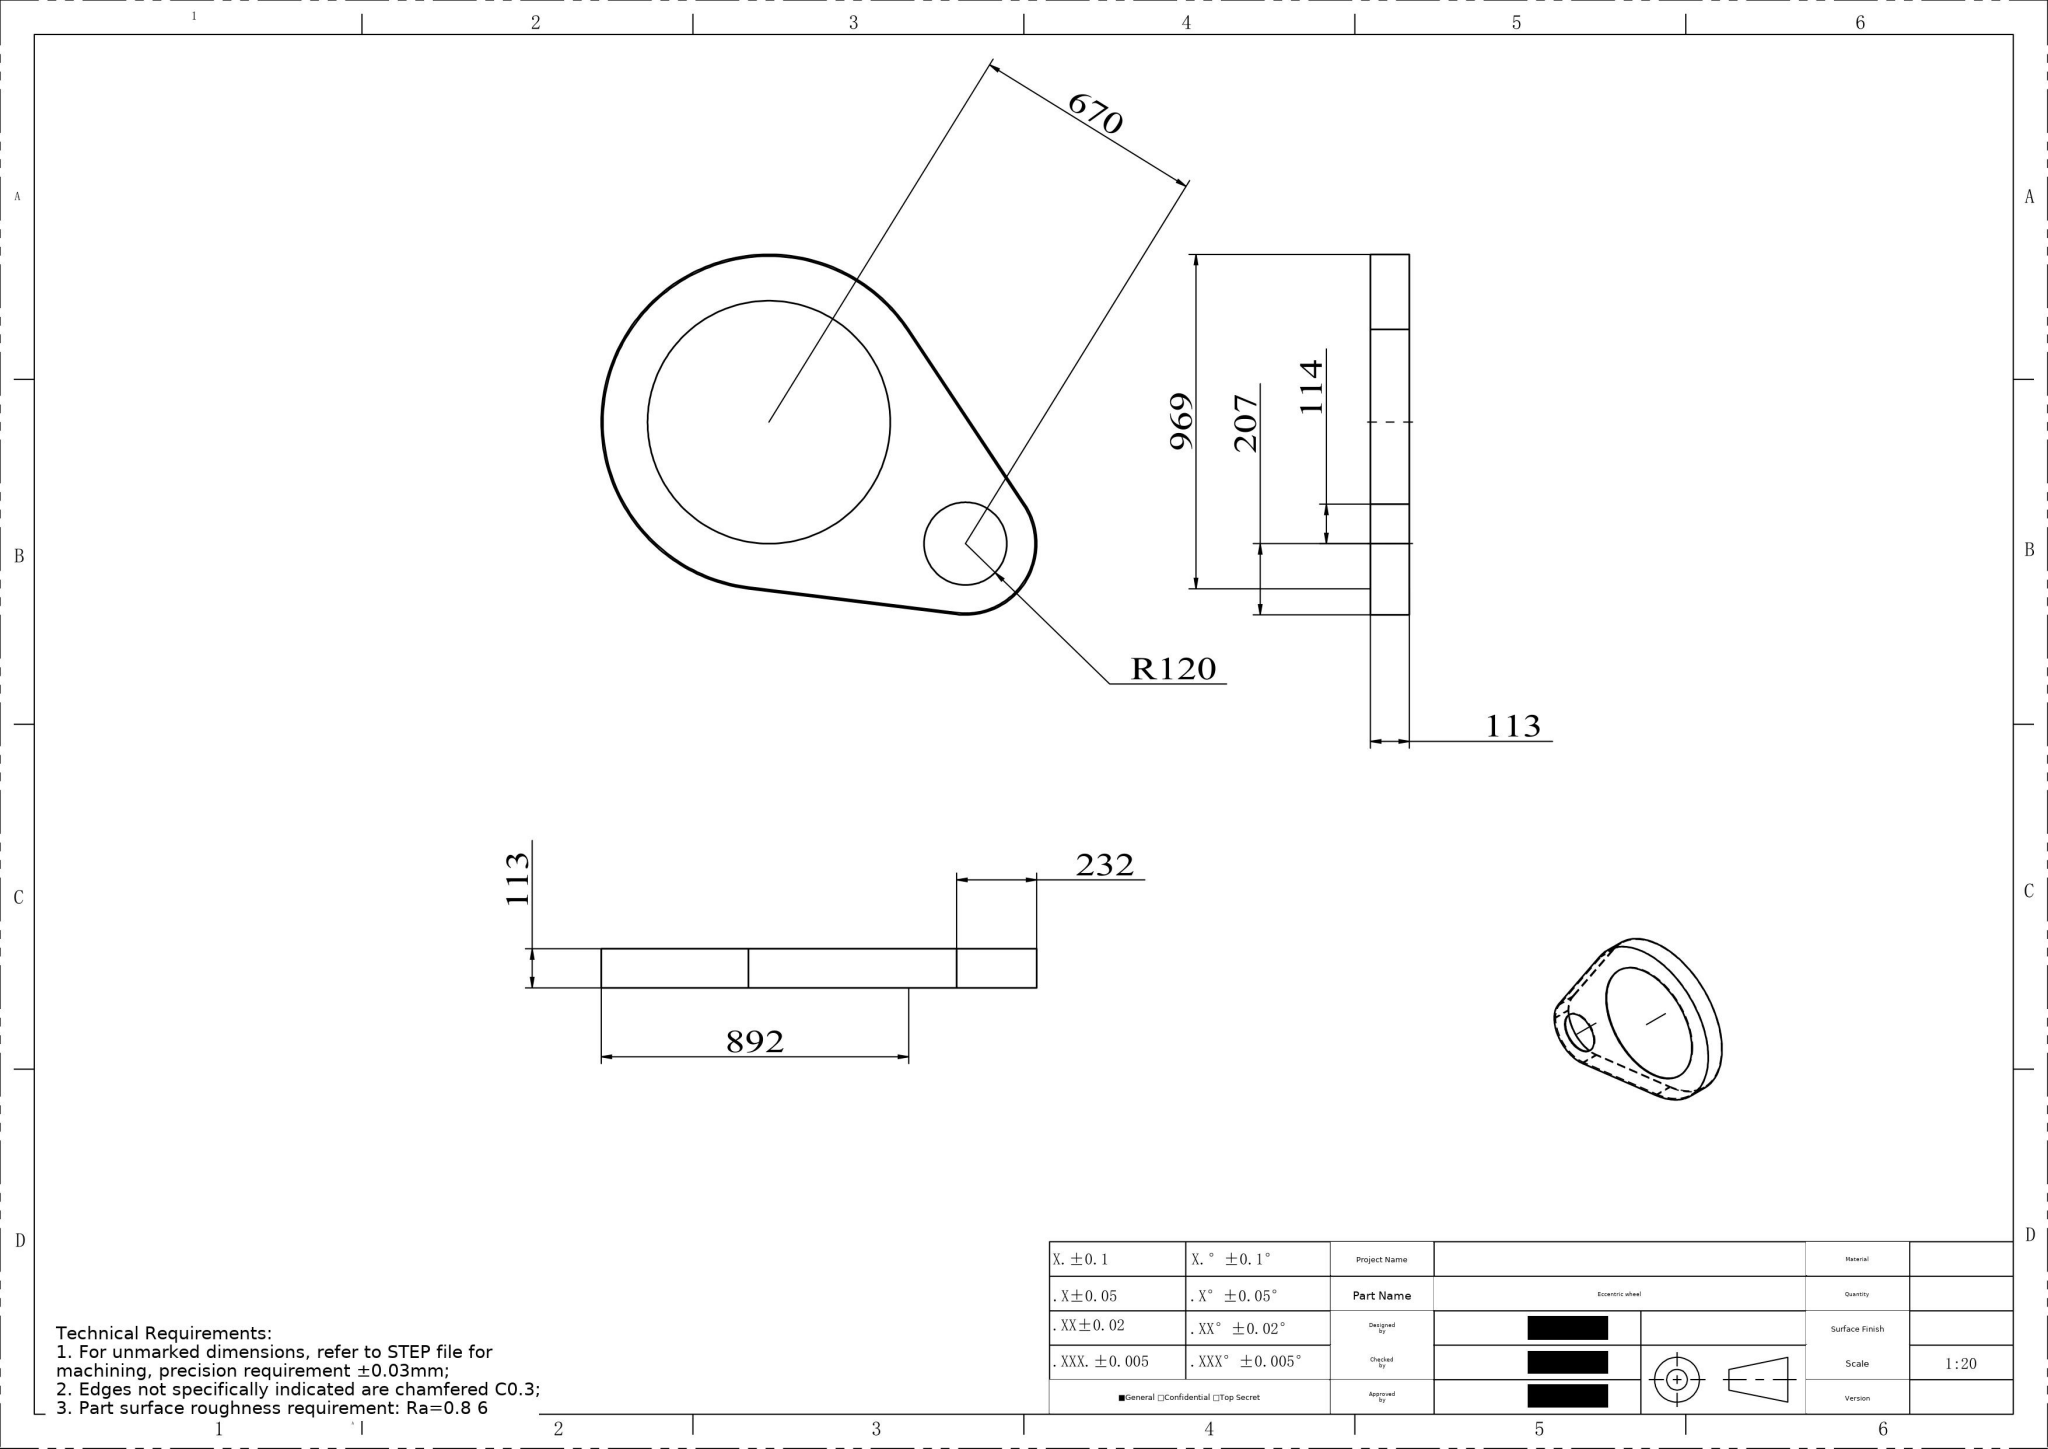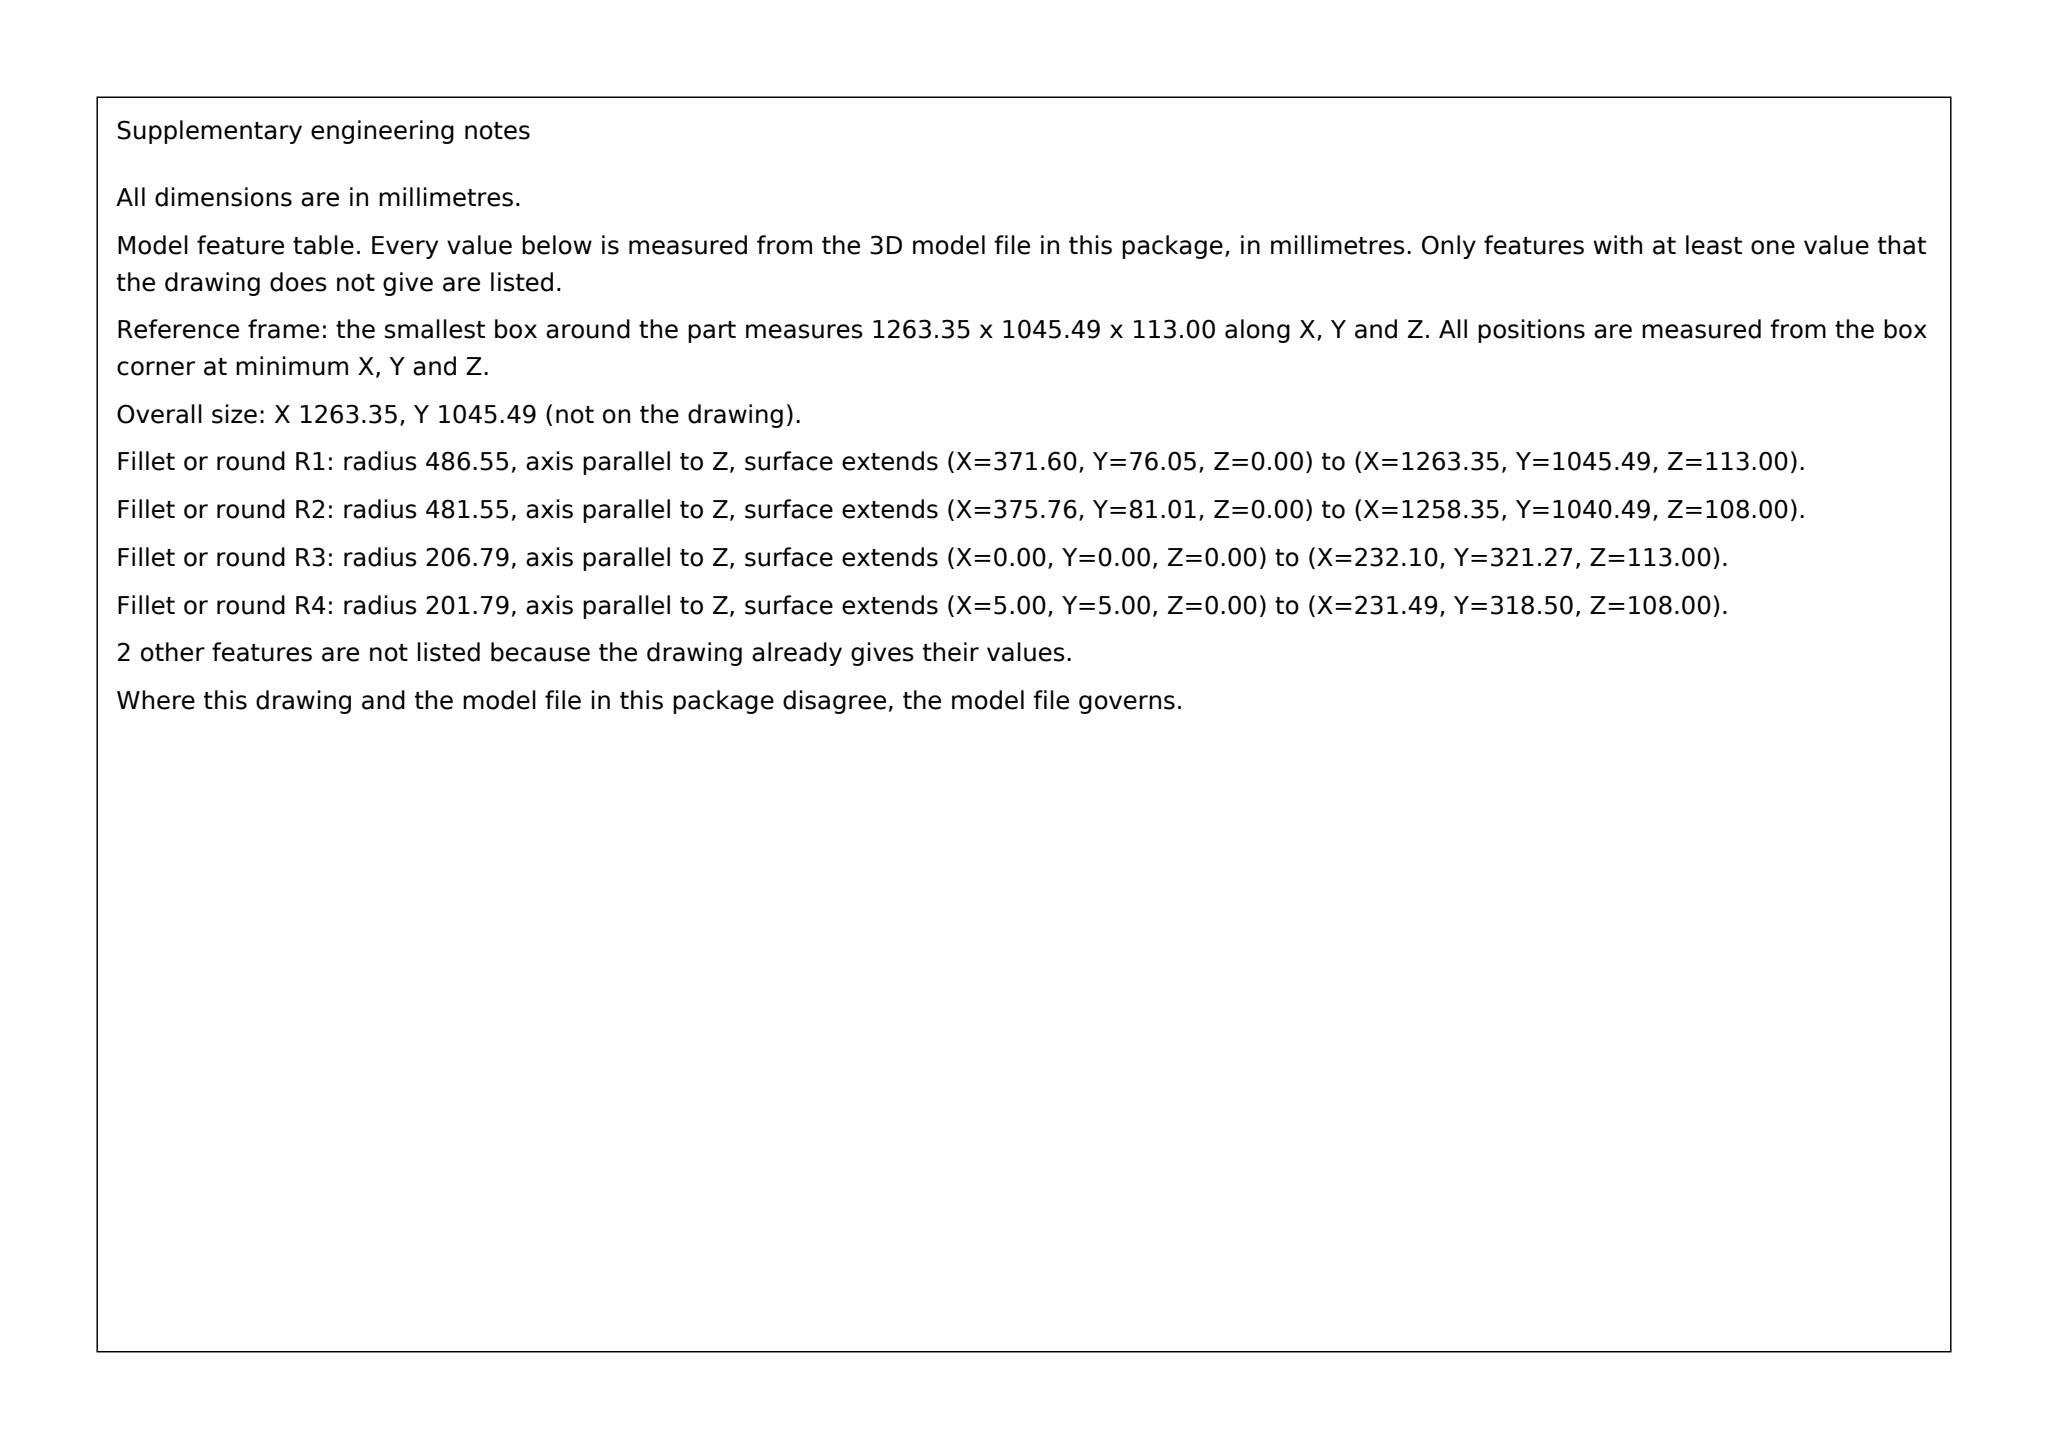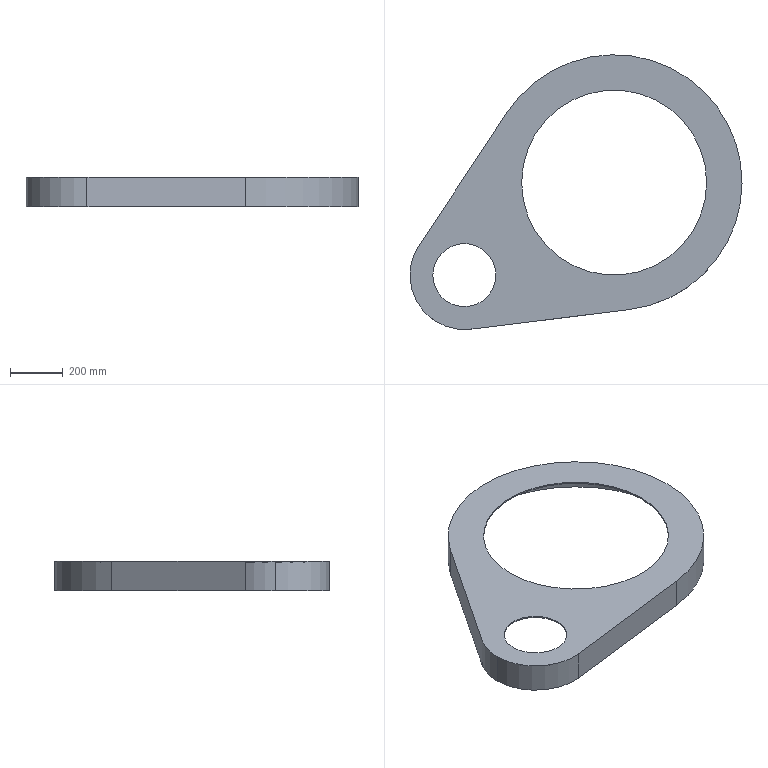Part | SolidWorks | mm | 1 solid | 17 faces | box 1263.35 x 1045.49 x 113 mm | volume 4506392 mm3 | cylinder 10 | plane 7 | commonest cylinder face diameters 240 x2 704 x2 403.589 x2 413.589 x2 963.102 x1 973.102 x1
STEP:
#1=CARTESIAN_POINT('',(-641.923,501.103,891.033));
#2=VERTEX_POINT('',#1);
#3=CARTESIAN_POINT('',(-641.923,501.103,886.033));
#4=VERTEX_POINT('',#3);
#5=CARTESIAN_POINT('',(-641.923,501.103,886.033));
#6=DIRECTION('',(0.,0.,-1.));
#7=VECTOR('',#6,1000.);
#8=LINE('',#5,#7);
#9=EDGE_CURVE('',#2,#4,#8,.T.);
#10=ORIENTED_EDGE('',*,*,#9,.F.);
#11=CARTESIAN_POINT('',(-881.923,501.103,891.033));
#12=VERTEX_POINT('',#11);
#13=CARTESIAN_POINT('',(-761.923,501.103,891.033));
#14=DIRECTION('',(0.,0.,-1.));
#15=DIRECTION('',(-1.,0.,0.));
#16=AXIS2_PLACEMENT_3D('',#13,#14,#15);
#17=CIRCLE('',#16,120.);
#18=EDGE_CURVE('',#12,#2,#17,.T.);
#19=ORIENTED_EDGE('',*,*,#18,.F.);
#20=CARTESIAN_POINT('',(-881.923,501.103,886.033));
#21=VERTEX_POINT('',#20);
#22=CARTESIAN_POINT('',(-881.923,501.103,886.033));
#23=DIRECTION('',(0.,0.,-1.));
#24=VECTOR('',#23,1000.);
#25=LINE('',#22,#24);
#26=EDGE_CURVE('',#12,#21,#25,.T.);
#27=ORIENTED_EDGE('',*,*,#26,.T.);
#28=CARTESIAN_POINT('',(-761.923,501.103,886.033));
#29=DIRECTION('',(0.,0.,-1.));
#30=DIRECTION('',(-1.,0.,0.));
#31=AXIS2_PLACEMENT_3D('',#28,#29,#30);
#32=CIRCLE('',#31,120.);
#33=EDGE_CURVE('',#21,#4,#32,.T.);
#34=ORIENTED_EDGE('',*,*,#33,.T.);
#35=EDGE_LOOP('',(#10,#19,#27,#34));
#36=FACE_OUTER_BOUND('',#35,.T.);
#37=CARTESIAN_POINT('',(-761.923,501.103,886.033));
#38=DIRECTION('',(0.,0.,-1.));
#39=DIRECTION('',(-1.,0.,0.));
#40=AXIS2_PLACEMENT_3D('',#37,#38,#39);
#41=CYLINDRICAL_SURFACE('',#40,120.);
#42=ADVANCED_FACE('',(#36),#41,.F.);
#43=CARTESIAN_POINT('',(160.077,853.249,891.033));
#44=VERTEX_POINT('',#43);
#45=CARTESIAN_POINT('',(160.077,853.249,886.033));
#46=VERTEX_POINT('',#45);
#47=CARTESIAN_POINT('',(160.077,853.249,886.033));
#48=DIRECTION('',(0.,0.,-1.));
#49=VECTOR('',#48,1000.);
#50=LINE('',#47,#49);
#51=EDGE_CURVE('',#44,#46,#50,.T.);
#52=ORIENTED_EDGE('',*,*,#51,.F.);
#53=CARTESIAN_POINT('',(-543.923,853.249,891.033));
#54=VERTEX_POINT('',#53);
#55=CARTESIAN_POINT('',(-191.923,853.249,891.033));
#56=DIRECTION('',(0.,0.,-1.));
#57=DIRECTION('',(-1.,0.,0.));
#58=AXIS2_PLACEMENT_3D('',#55,#56,#57);
#59=CIRCLE('',#58,352.);
#60=EDGE_CURVE('',#54,#44,#59,.T.);
#61=ORIENTED_EDGE('',*,*,#60,.F.);
#62=CARTESIAN_POINT('',(-543.923,853.249,886.033));
#63=VERTEX_POINT('',#62);
#64=CARTESIAN_POINT('',(-543.923,853.249,886.033));
#65=DIRECTION('',(0.,0.,-1.));
#66=VECTOR('',#65,1000.);
#67=LINE('',#64,#66);
#68=EDGE_CURVE('',#54,#63,#67,.T.);
#69=ORIENTED_EDGE('',*,*,#68,.T.);
#70=CARTESIAN_POINT('',(-191.923,853.249,886.033));
#71=DIRECTION('',(0.,0.,-1.));
#72=DIRECTION('',(-1.,0.,0.));
#73=AXIS2_PLACEMENT_3D('',#70,#71,#72);
#74=CIRCLE('',#73,352.);
#75=EDGE_CURVE('',#63,#46,#74,.T.);
#76=ORIENTED_EDGE('',*,*,#75,.T.);
#77=EDGE_LOOP('',(#52,#61,#69,#76));
#78=FACE_OUTER_BOUND('',#77,.T.);
#79=CARTESIAN_POINT('',(-191.923,853.249,886.033));
#80=DIRECTION('',(0.,0.,-1.));
#81=DIRECTION('',(-1.,0.,0.));
#82=AXIS2_PLACEMENT_3D('',#79,#80,#81);
#83=CYLINDRICAL_SURFACE('',#82,352.);
#84=ADVANCED_FACE('',(#78),#83,.F.);
#85=ORIENTED_EDGE('',*,*,#75,.F.);
#86=CARTESIAN_POINT('',(-191.923,853.249,886.033));
#87=DIRECTION('',(0.,0.,-1.));
#88=DIRECTION('',(-1.,0.,0.));
#89=AXIS2_PLACEMENT_3D('',#86,#87,#88);
#90=CIRCLE('',#89,352.);
#91=EDGE_CURVE('',#46,#63,#90,.T.);
#92=ORIENTED_EDGE('',*,*,#91,.F.);
#93=EDGE_LOOP('',(#85,#92));
#94=FACE_BOUND('',#93,.T.);
#95=ORIENTED_EDGE('',*,*,#33,.F.);
#96=CARTESIAN_POINT('',(-761.923,501.103,886.033));
#97=DIRECTION('',(0.,0.,-1.));
#98=DIRECTION('',(-1.,0.,0.));
#99=AXIS2_PLACEMENT_3D('',#96,#97,#98);
#100=CIRCLE('',#99,120.);
#101=EDGE_CURVE('',#4,#21,#100,.T.);
#102=ORIENTED_EDGE('',*,*,#101,.F.);
#103=EDGE_LOOP('',(#95,#102));
#104=FACE_BOUND('',#103,.T.);
#105=CARTESIAN_POINT('',(-592.958,1119.824,886.033));
#106=VERTEX_POINT('',#105);
#107=CARTESIAN_POINT('',(-133.002,375.316,886.033));
#108=VERTEX_POINT('',#107);
#109=CARTESIAN_POINT('',(-191.923,853.249,886.033));
#110=DIRECTION('',(0.,0.,-1.));
#111=DIRECTION('',(-1.,0.,0.));
#112=AXIS2_PLACEMENT_3D('',#109,#110,#111);
#113=CIRCLE('',#112,481.551);
#114=EDGE_CURVE('',#106,#108,#113,.T.);
#115=ORIENTED_EDGE('',*,*,#114,.T.);
#116=CARTESIAN_POINT('',(-737.232,300.825,886.033));
#117=VERTEX_POINT('',#116);
#118=CARTESIAN_POINT('',(-133.002,375.316,886.033));
#119=DIRECTION('',(-0.9925,-0.1224,0.));
#120=VECTOR('',#119,1000.);
#121=LINE('',#118,#120);
#122=EDGE_CURVE('',#108,#117,#121,.T.);
#123=ORIENTED_EDGE('',*,*,#122,.T.);
#124=CARTESIAN_POINT('',(-963.718,501.103,886.033));
#125=VERTEX_POINT('',#124);
#126=CARTESIAN_POINT('',(-761.923,501.103,886.033));
#127=DIRECTION('',(0.,0.,-1.));
#128=DIRECTION('',(-1.,0.,0.));
#129=AXIS2_PLACEMENT_3D('',#126,#127,#128);
#130=CIRCLE('',#129,201.795);
#131=EDGE_CURVE('',#117,#125,#130,.T.);
#132=ORIENTED_EDGE('',*,*,#131,.T.);
#133=CARTESIAN_POINT('',(-929.977,612.812,886.033));
#134=VERTEX_POINT('',#133);
#135=CARTESIAN_POINT('',(-761.923,501.103,886.033));
#136=DIRECTION('',(0.,0.,-1.));
#137=DIRECTION('',(-1.,0.,0.));
#138=AXIS2_PLACEMENT_3D('',#135,#136,#137);
#139=CIRCLE('',#138,201.795);
#140=EDGE_CURVE('',#125,#134,#139,.T.);
#141=ORIENTED_EDGE('',*,*,#140,.T.);
#142=CARTESIAN_POINT('',(-929.977,612.812,886.033));
#143=DIRECTION('',(0.5536,0.8328,0.));
#144=VECTOR('',#143,1000.);
#145=LINE('',#142,#144);
#146=EDGE_CURVE('',#134,#106,#145,.T.);
#147=ORIENTED_EDGE('',*,*,#146,.T.);
#148=EDGE_LOOP('',(#115,#123,#132,#141,#147));
#149=FACE_OUTER_BOUND('',#148,.T.);
#150=CARTESIAN_POINT('',(-191.923,853.249,886.033));
#151=DIRECTION('',(0.,0.,-1.));
#152=DIRECTION('',(0.,-1.,0.));
#153=AXIS2_PLACEMENT_3D('',#150,#151,#152);
#154=PLANE('',#153);
#155=ADVANCED_FACE('',(#94,#104,#149),#154,.T.);
#156=CARTESIAN_POINT('',(-133.002,375.316,778.033));
#157=VERTEX_POINT('',#156);
#158=CARTESIAN_POINT('',(-737.232,300.825,778.033));
#159=VERTEX_POINT('',#158);
#160=CARTESIAN_POINT('',(-133.002,375.316,778.033));
#161=DIRECTION('',(-0.9925,-0.1224,0.));
#162=VECTOR('',#161,1000.);
#163=LINE('',#160,#162);
#164=EDGE_CURVE('',#157,#159,#163,.T.);
#165=ORIENTED_EDGE('',*,*,#164,.T.);
#166=CARTESIAN_POINT('',(-737.232,300.825,886.033));
#167=DIRECTION('',(0.,0.,-1.));
#168=VECTOR('',#167,1000.);
#169=LINE('',#166,#168);
#170=EDGE_CURVE('',#117,#159,#169,.T.);
#171=ORIENTED_EDGE('',*,*,#170,.F.);
#172=ORIENTED_EDGE('',*,*,#122,.F.);
#173=CARTESIAN_POINT('',(-133.002,375.316,886.033));
#174=DIRECTION('',(0.,0.,-1.));
#175=VECTOR('',#174,1000.);
#176=LINE('',#173,#175);
#177=EDGE_CURVE('',#108,#157,#176,.T.);
#178=ORIENTED_EDGE('',*,*,#177,.T.);
#179=EDGE_LOOP('',(#165,#171,#172,#178));
#180=FACE_OUTER_BOUND('',#179,.T.);
#181=CARTESIAN_POINT('',(-133.002,375.316,886.033));
#182=DIRECTION('',(0.1224,-0.9925,0.));
#183=DIRECTION('',(0.,0.,-1.));
#184=AXIS2_PLACEMENT_3D('',#181,#182,#183);
#185=PLANE('',#184);
#186=ADVANCED_FACE('',(#180),#185,.F.);
#187=CARTESIAN_POINT('',(-963.718,501.103,778.033));
#188=VERTEX_POINT('',#187);
#189=CARTESIAN_POINT('',(-963.718,501.103,886.033));
#190=DIRECTION('',(0.,0.,-1.));
#191=VECTOR('',#190,1000.);
#192=LINE('',#189,#191);
#193=EDGE_CURVE('',#125,#188,#192,.T.);
#194=ORIENTED_EDGE('',*,*,#193,.F.);
#195=ORIENTED_EDGE('',*,*,#131,.F.);
#196=ORIENTED_EDGE('',*,*,#170,.T.);
#197=CARTESIAN_POINT('',(-761.923,501.103,778.033));
#198=DIRECTION('',(0.,0.,-1.));
#199=DIRECTION('',(-1.,0.,0.));
#200=AXIS2_PLACEMENT_3D('',#197,#198,#199);
#201=CIRCLE('',#200,201.795);
#202=EDGE_CURVE('',#159,#188,#201,.T.);
#203=ORIENTED_EDGE('',*,*,#202,.T.);
#204=EDGE_LOOP('',(#194,#195,#196,#203));
#205=FACE_OUTER_BOUND('',#204,.T.);
#206=CARTESIAN_POINT('',(-761.923,501.103,886.033));
#207=DIRECTION('',(0.,0.,-1.));
#208=DIRECTION('',(-1.,0.,0.));
#209=AXIS2_PLACEMENT_3D('',#206,#207,#208);
#210=CYLINDRICAL_SURFACE('',#209,201.795);
#211=ADVANCED_FACE('',(#205),#210,.F.);
#212=CARTESIAN_POINT('',(-929.977,612.812,778.033));
#213=VERTEX_POINT('',#212);
#214=CARTESIAN_POINT('',(-592.958,1119.824,778.033));
#215=VERTEX_POINT('',#214);
#216=CARTESIAN_POINT('',(-929.977,612.812,778.033));
#217=DIRECTION('',(0.5536,0.8328,0.));
#218=VECTOR('',#217,1000.);
#219=LINE('',#216,#218);
#220=EDGE_CURVE('',#213,#215,#219,.T.);
#221=ORIENTED_EDGE('',*,*,#220,.T.);
#222=CARTESIAN_POINT('',(-592.958,1119.824,886.033));
#223=DIRECTION('',(0.,0.,-1.));
#224=VECTOR('',#223,1000.);
#225=LINE('',#222,#224);
#226=EDGE_CURVE('',#106,#215,#225,.T.);
#227=ORIENTED_EDGE('',*,*,#226,.F.);
#228=ORIENTED_EDGE('',*,*,#146,.F.);
#229=CARTESIAN_POINT('',(-929.977,612.812,886.033));
#230=DIRECTION('',(0.,0.,-1.));
#231=VECTOR('',#230,1000.);
#232=LINE('',#229,#231);
#233=EDGE_CURVE('',#134,#213,#232,.T.);
#234=ORIENTED_EDGE('',*,*,#233,.T.);
#235=EDGE_LOOP('',(#221,#227,#228,#234));
#236=FACE_OUTER_BOUND('',#235,.T.);
#237=CARTESIAN_POINT('',(-929.977,612.812,886.033));
#238=DIRECTION('',(-0.8328,0.5536,0.));
#239=DIRECTION('',(0.,0.,1.));
#240=AXIS2_PLACEMENT_3D('',#237,#238,#239);
#241=PLANE('',#240);
#242=ADVANCED_FACE('',(#236),#241,.F.);
#243=CARTESIAN_POINT('',(-191.923,853.249,778.033));
#244=DIRECTION('',(0.,0.,-1.));
#245=DIRECTION('',(-1.,0.,0.));
#246=AXIS2_PLACEMENT_3D('',#243,#244,#245);
#247=CIRCLE('',#246,481.551);
#248=EDGE_CURVE('',#215,#157,#247,.T.);
#249=ORIENTED_EDGE('',*,*,#248,.T.);
#250=ORIENTED_EDGE('',*,*,#177,.F.);
#251=ORIENTED_EDGE('',*,*,#114,.F.);
#252=ORIENTED_EDGE('',*,*,#226,.T.);
#253=EDGE_LOOP('',(#249,#250,#251,#252));
#254=FACE_OUTER_BOUND('',#253,.T.);
#255=CARTESIAN_POINT('',(-191.923,853.249,886.033));
#256=DIRECTION('',(0.,0.,-1.));
#257=DIRECTION('',(-1.,0.,0.));
#258=AXIS2_PLACEMENT_3D('',#255,#256,#257);
#259=CYLINDRICAL_SURFACE('',#258,481.551);
#260=ADVANCED_FACE('',(#254),#259,.F.);
#261=ORIENTED_EDGE('',*,*,#248,.F.);
#262=ORIENTED_EDGE('',*,*,#220,.F.);
#263=CARTESIAN_POINT('',(-761.923,501.103,778.033));
#264=DIRECTION('',(0.,0.,-1.));
#265=DIRECTION('',(-1.,0.,0.));
#266=AXIS2_PLACEMENT_3D('',#263,#264,#265);
#267=CIRCLE('',#266,201.795);
#268=EDGE_CURVE('',#188,#213,#267,.T.);
#269=ORIENTED_EDGE('',*,*,#268,.F.);
#270=ORIENTED_EDGE('',*,*,#202,.F.);
#271=ORIENTED_EDGE('',*,*,#164,.F.);
#272=EDGE_LOOP('',(#261,#262,#269,#270,#271));
#273=FACE_BOUND('',#272,.T.);
#274=CARTESIAN_POINT('',(-597.122,1122.591,778.033));
#275=VERTEX_POINT('',#274);
#276=CARTESIAN_POINT('',(-132.39,370.354,778.033));
#277=VERTEX_POINT('',#276);
#278=CARTESIAN_POINT('',(-191.923,853.249,778.033));
#279=DIRECTION('',(0.,0.,-1.));
#280=DIRECTION('',(-1.,0.,0.));
#281=AXIS2_PLACEMENT_3D('',#278,#279,#280);
#282=CIRCLE('',#281,486.551);
#283=EDGE_CURVE('',#275,#277,#282,.T.);
#284=ORIENTED_EDGE('',*,*,#283,.T.);
#285=CARTESIAN_POINT('',(-736.62,295.862,778.033));
#286=VERTEX_POINT('',#285);
#287=CARTESIAN_POINT('',(-132.39,370.354,778.033));
#288=DIRECTION('',(-0.9925,-0.1224,0.));
#289=VECTOR('',#288,1000.);
#290=LINE('',#287,#289);
#291=EDGE_CURVE('',#277,#286,#290,.T.);
#292=ORIENTED_EDGE('',*,*,#291,.T.);
#293=CARTESIAN_POINT('',(-968.718,501.103,778.033));
#294=VERTEX_POINT('',#293);
#295=CARTESIAN_POINT('',(-761.923,501.103,778.033));
#296=DIRECTION('',(0.,0.,-1.));
#297=DIRECTION('',(-1.,0.,0.));
#298=AXIS2_PLACEMENT_3D('',#295,#296,#297);
#299=CIRCLE('',#298,206.795);
#300=EDGE_CURVE('',#286,#294,#299,.T.);
#301=ORIENTED_EDGE('',*,*,#300,.T.);
#302=CARTESIAN_POINT('',(-934.141,615.58,778.033));
#303=VERTEX_POINT('',#302);
#304=CARTESIAN_POINT('',(-761.923,501.103,778.033));
#305=DIRECTION('',(0.,0.,-1.));
#306=DIRECTION('',(-1.,0.,0.));
#307=AXIS2_PLACEMENT_3D('',#304,#305,#306);
#308=CIRCLE('',#307,206.795);
#309=EDGE_CURVE('',#294,#303,#308,.T.);
#310=ORIENTED_EDGE('',*,*,#309,.T.);
#311=CARTESIAN_POINT('',(-934.141,615.58,778.033));
#312=DIRECTION('',(0.5536,0.8328,0.));
#313=VECTOR('',#312,1000.);
#314=LINE('',#311,#313);
#315=EDGE_CURVE('',#303,#275,#314,.T.);
#316=ORIENTED_EDGE('',*,*,#315,.T.);
#317=EDGE_LOOP('',(#284,#292,#301,#310,#316));
#318=FACE_OUTER_BOUND('',#317,.T.);
#319=CARTESIAN_POINT('',(-191.923,853.249,778.033));
#320=DIRECTION('',(0.,0.,-1.));
#321=DIRECTION('',(0.,-1.,0.));
#322=AXIS2_PLACEMENT_3D('',#319,#320,#321);
#323=PLANE('',#322);
#324=ADVANCED_FACE('',(#273,#318),#323,.T.);
#325=ORIENTED_EDGE('',*,*,#60,.T.);
#326=CARTESIAN_POINT('',(-191.923,853.249,891.033));
#327=DIRECTION('',(0.,0.,-1.));
#328=DIRECTION('',(-1.,0.,0.));
#329=AXIS2_PLACEMENT_3D('',#326,#327,#328);
#330=CIRCLE('',#329,352.);
#331=EDGE_CURVE('',#44,#54,#330,.T.);
#332=ORIENTED_EDGE('',*,*,#331,.T.);
#333=EDGE_LOOP('',(#325,#332));
#334=FACE_BOUND('',#333,.T.);
#335=ORIENTED_EDGE('',*,*,#18,.T.);
#336=CARTESIAN_POINT('',(-761.923,501.103,891.033));
#337=DIRECTION('',(0.,0.,-1.));
#338=DIRECTION('',(-1.,0.,0.));
#339=AXIS2_PLACEMENT_3D('',#336,#337,#338);
#340=CIRCLE('',#339,120.);
#341=EDGE_CURVE('',#2,#12,#340,.T.);
#342=ORIENTED_EDGE('',*,*,#341,.T.);
#343=EDGE_LOOP('',(#335,#342));
#344=FACE_BOUND('',#343,.T.);
#345=CARTESIAN_POINT('',(-597.122,1122.591,891.033));
#346=VERTEX_POINT('',#345);
#347=CARTESIAN_POINT('',(-132.39,370.354,891.033));
#348=VERTEX_POINT('',#347);
#349=CARTESIAN_POINT('',(-191.923,853.249,891.033));
#350=DIRECTION('',(0.,0.,-1.));
#351=DIRECTION('',(-1.,0.,0.));
#352=AXIS2_PLACEMENT_3D('',#349,#350,#351);
#353=CIRCLE('',#352,486.551);
#354=EDGE_CURVE('',#346,#348,#353,.T.);
#355=ORIENTED_EDGE('',*,*,#354,.F.);
#356=CARTESIAN_POINT('',(-934.141,615.58,891.033));
#357=VERTEX_POINT('',#356);
#358=CARTESIAN_POINT('',(-934.141,615.58,891.033));
#359=DIRECTION('',(0.5536,0.8328,0.));
#360=VECTOR('',#359,1000.);
#361=LINE('',#358,#360);
#362=EDGE_CURVE('',#357,#346,#361,.T.);
#363=ORIENTED_EDGE('',*,*,#362,.F.);
#364=CARTESIAN_POINT('',(-968.718,501.103,891.033));
#365=VERTEX_POINT('',#364);
#366=CARTESIAN_POINT('',(-761.923,501.103,891.033));
#367=DIRECTION('',(0.,0.,-1.));
#368=DIRECTION('',(-1.,0.,0.));
#369=AXIS2_PLACEMENT_3D('',#366,#367,#368);
#370=CIRCLE('',#369,206.795);
#371=EDGE_CURVE('',#365,#357,#370,.T.);
#372=ORIENTED_EDGE('',*,*,#371,.F.);
#373=CARTESIAN_POINT('',(-736.62,295.862,891.033));
#374=VERTEX_POINT('',#373);
#375=CARTESIAN_POINT('',(-761.923,501.103,891.033));
#376=DIRECTION('',(0.,0.,-1.));
#377=DIRECTION('',(-1.,0.,0.));
#378=AXIS2_PLACEMENT_3D('',#375,#376,#377);
#379=CIRCLE('',#378,206.795);
#380=EDGE_CURVE('',#374,#365,#379,.T.);
#381=ORIENTED_EDGE('',*,*,#380,.F.);
#382=CARTESIAN_POINT('',(-132.39,370.354,891.033));
#383=DIRECTION('',(-0.9925,-0.1224,0.));
#384=VECTOR('',#383,1000.);
#385=LINE('',#382,#384);
#386=EDGE_CURVE('',#348,#374,#385,.T.);
#387=ORIENTED_EDGE('',*,*,#386,.F.);
#388=EDGE_LOOP('',(#355,#363,#372,#381,#387));
#389=FACE_OUTER_BOUND('',#388,.T.);
#390=CARTESIAN_POINT('',(-191.923,853.249,891.033));
#391=DIRECTION('',(0.,0.,-1.));
#392=DIRECTION('',(0.,-1.,0.));
#393=AXIS2_PLACEMENT_3D('',#390,#391,#392);
#394=PLANE('',#393);
#395=ADVANCED_FACE('',(#334,#344,#389),#394,.F.);
#396=ORIENTED_EDGE('',*,*,#291,.F.);
#397=CARTESIAN_POINT('',(-132.39,370.354,891.033));
#398=DIRECTION('',(0.,0.,-1.));
#399=VECTOR('',#398,1000.);
#400=LINE('',#397,#399);
#401=EDGE_CURVE('',#348,#277,#400,.T.);
#402=ORIENTED_EDGE('',*,*,#401,.F.);
#403=ORIENTED_EDGE('',*,*,#386,.T.);
#404=CARTESIAN_POINT('',(-736.62,295.862,891.033));
#405=DIRECTION('',(0.,0.,-1.));
#406=VECTOR('',#405,1000.);
#407=LINE('',#404,#406);
#408=EDGE_CURVE('',#374,#286,#407,.T.);
#409=ORIENTED_EDGE('',*,*,#408,.T.);
#410=EDGE_LOOP('',(#396,#402,#403,#409));
#411=FACE_OUTER_BOUND('',#410,.T.);
#412=CARTESIAN_POINT('',(-132.39,370.354,891.033));
#413=DIRECTION('',(0.1224,-0.9925,0.));
#414=DIRECTION('',(0.,0.,-1.));
#415=AXIS2_PLACEMENT_3D('',#412,#413,#414);
#416=PLANE('',#415);
#417=ADVANCED_FACE('',(#411),#416,.T.);
#418=CARTESIAN_POINT('',(-968.718,501.103,891.033));
#419=DIRECTION('',(0.,0.,-1.));
#420=VECTOR('',#419,1000.);
#421=LINE('',#418,#420);
#422=EDGE_CURVE('',#365,#294,#421,.T.);
#423=ORIENTED_EDGE('',*,*,#422,.F.);
#424=ORIENTED_EDGE('',*,*,#371,.T.);
#425=CARTESIAN_POINT('',(-934.141,615.58,891.033));
#426=DIRECTION('',(0.,0.,-1.));
#427=VECTOR('',#426,1000.);
#428=LINE('',#425,#427);
#429=EDGE_CURVE('',#357,#303,#428,.T.);
#430=ORIENTED_EDGE('',*,*,#429,.T.);
#431=ORIENTED_EDGE('',*,*,#309,.F.);
#432=EDGE_LOOP('',(#423,#424,#430,#431));
#433=FACE_OUTER_BOUND('',#432,.T.);
#434=CARTESIAN_POINT('',(-761.923,501.103,891.033));
#435=DIRECTION('',(0.,0.,-1.));
#436=DIRECTION('',(-1.,0.,0.));
#437=AXIS2_PLACEMENT_3D('',#434,#435,#436);
#438=CYLINDRICAL_SURFACE('',#437,206.795);
#439=ADVANCED_FACE('',(#433),#438,.T.);
#440=ORIENTED_EDGE('',*,*,#315,.F.);
#441=ORIENTED_EDGE('',*,*,#429,.F.);
#442=ORIENTED_EDGE('',*,*,#362,.T.);
#443=CARTESIAN_POINT('',(-597.122,1122.591,891.033));
#444=DIRECTION('',(0.,0.,-1.));
#445=VECTOR('',#444,1000.);
#446=LINE('',#443,#445);
#447=EDGE_CURVE('',#346,#275,#446,.T.);
#448=ORIENTED_EDGE('',*,*,#447,.T.);
#449=EDGE_LOOP('',(#440,#441,#442,#448));
#450=FACE_OUTER_BOUND('',#449,.T.);
#451=CARTESIAN_POINT('',(-934.141,615.58,891.033));
#452=DIRECTION('',(-0.8328,0.5536,0.));
#453=DIRECTION('',(0.,0.,1.));
#454=AXIS2_PLACEMENT_3D('',#451,#452,#453);
#455=PLANE('',#454);
#456=ADVANCED_FACE('',(#450),#455,.T.);
#457=ORIENTED_EDGE('',*,*,#283,.F.);
#458=ORIENTED_EDGE('',*,*,#447,.F.);
#459=ORIENTED_EDGE('',*,*,#354,.T.);
#460=ORIENTED_EDGE('',*,*,#401,.T.);
#461=EDGE_LOOP('',(#457,#458,#459,#460));
#462=FACE_OUTER_BOUND('',#461,.T.);
#463=CARTESIAN_POINT('',(-191.923,853.249,891.033));
#464=DIRECTION('',(0.,0.,-1.));
#465=DIRECTION('',(-1.,0.,0.));
#466=AXIS2_PLACEMENT_3D('',#463,#464,#465);
#467=CYLINDRICAL_SURFACE('',#466,486.551);
#468=ADVANCED_FACE('',(#462),#467,.T.);
#469=ORIENTED_EDGE('',*,*,#380,.T.);
#470=ORIENTED_EDGE('',*,*,#422,.T.);
#471=ORIENTED_EDGE('',*,*,#300,.F.);
#472=ORIENTED_EDGE('',*,*,#408,.F.);
#473=EDGE_LOOP('',(#469,#470,#471,#472));
#474=FACE_OUTER_BOUND('',#473,.T.);
#475=CARTESIAN_POINT('',(-761.923,501.103,891.033));
#476=DIRECTION('',(0.,0.,-1.));
#477=DIRECTION('',(-1.,0.,0.));
#478=AXIS2_PLACEMENT_3D('',#475,#476,#477);
#479=CYLINDRICAL_SURFACE('',#478,206.795);
#480=ADVANCED_FACE('',(#474),#479,.T.);
#481=ORIENTED_EDGE('',*,*,#140,.F.);
#482=ORIENTED_EDGE('',*,*,#193,.T.);
#483=ORIENTED_EDGE('',*,*,#268,.T.);
#484=ORIENTED_EDGE('',*,*,#233,.F.);
#485=EDGE_LOOP('',(#481,#482,#483,#484));
#486=FACE_OUTER_BOUND('',#485,.T.);
#487=CARTESIAN_POINT('',(-761.923,501.103,886.033));
#488=DIRECTION('',(0.,0.,-1.));
#489=DIRECTION('',(-1.,0.,0.));
#490=AXIS2_PLACEMENT_3D('',#487,#488,#489);
#491=CYLINDRICAL_SURFACE('',#490,201.795);
#492=ADVANCED_FACE('',(#486),#491,.F.);
#493=ORIENTED_EDGE('',*,*,#331,.F.);
#494=ORIENTED_EDGE('',*,*,#51,.T.);
#495=ORIENTED_EDGE('',*,*,#91,.T.);
#496=ORIENTED_EDGE('',*,*,#68,.F.);
#497=EDGE_LOOP('',(#493,#494,#495,#496));
#498=FACE_OUTER_BOUND('',#497,.T.);
#499=CARTESIAN_POINT('',(-191.923,853.249,886.033));
#500=DIRECTION('',(0.,0.,-1.));
#501=DIRECTION('',(-1.,0.,0.));
#502=AXIS2_PLACEMENT_3D('',#499,#500,#501);
#503=CYLINDRICAL_SURFACE('',#502,352.);
#504=ADVANCED_FACE('',(#498),#503,.F.);
#505=ORIENTED_EDGE('',*,*,#341,.F.);
#506=ORIENTED_EDGE('',*,*,#9,.T.);
#507=ORIENTED_EDGE('',*,*,#101,.T.);
#508=ORIENTED_EDGE('',*,*,#26,.F.);
#509=EDGE_LOOP('',(#505,#506,#507,#508));
#510=FACE_OUTER_BOUND('',#509,.T.);
#511=CARTESIAN_POINT('',(-761.923,501.103,886.033));
#512=DIRECTION('',(0.,0.,-1.));
#513=DIRECTION('',(-1.,0.,0.));
#514=AXIS2_PLACEMENT_3D('',#511,#512,#513);
#515=CYLINDRICAL_SURFACE('',#514,120.);
#516=ADVANCED_FACE('',(#510),#515,.F.);
#517=CLOSED_SHELL('',(#42,#84,#155,#186,#211,#242,#260,#324,#395,#417,#439,#456,#468,#480,#492,#504,#516));
#518=MANIFOLD_SOLID_BREP('',#517);
#519=CARTESIAN_POINT('',(0.,0.,0.));
#520=DIRECTION('',(0.,0.,1.));
#521=DIRECTION('',(1.,0.,0.));
#522=AXIS2_PLACEMENT_3D('',#519,#520,#521);
#523=(LENGTH_UNIT()NAMED_UNIT(*)SI_UNIT(.MILLI.,.METRE.));
#524=UNCERTAINTY_MEASURE_WITH_UNIT(LENGTH_MEASURE(0.00001),#523,'','');
#525=(NAMED_UNIT(*)PLANE_ANGLE_UNIT()SI_UNIT($,.RADIAN.));
#526=(NAMED_UNIT(*)SI_UNIT($,.STERADIAN.)SOLID_ANGLE_UNIT());
#527=(GEOMETRIC_REPRESENTATION_CONTEXT(3)GLOBAL_UNCERTAINTY_ASSIGNED_CONTEXT((#524))GLOBAL_UNIT_ASSIGNED_CONTEXT((#523,#525,#526))REPRESENTATION_CONTEXT('',''));
#528=ADVANCED_BREP_SHAPE_REPRESENTATION('',(#518,#522),#527);